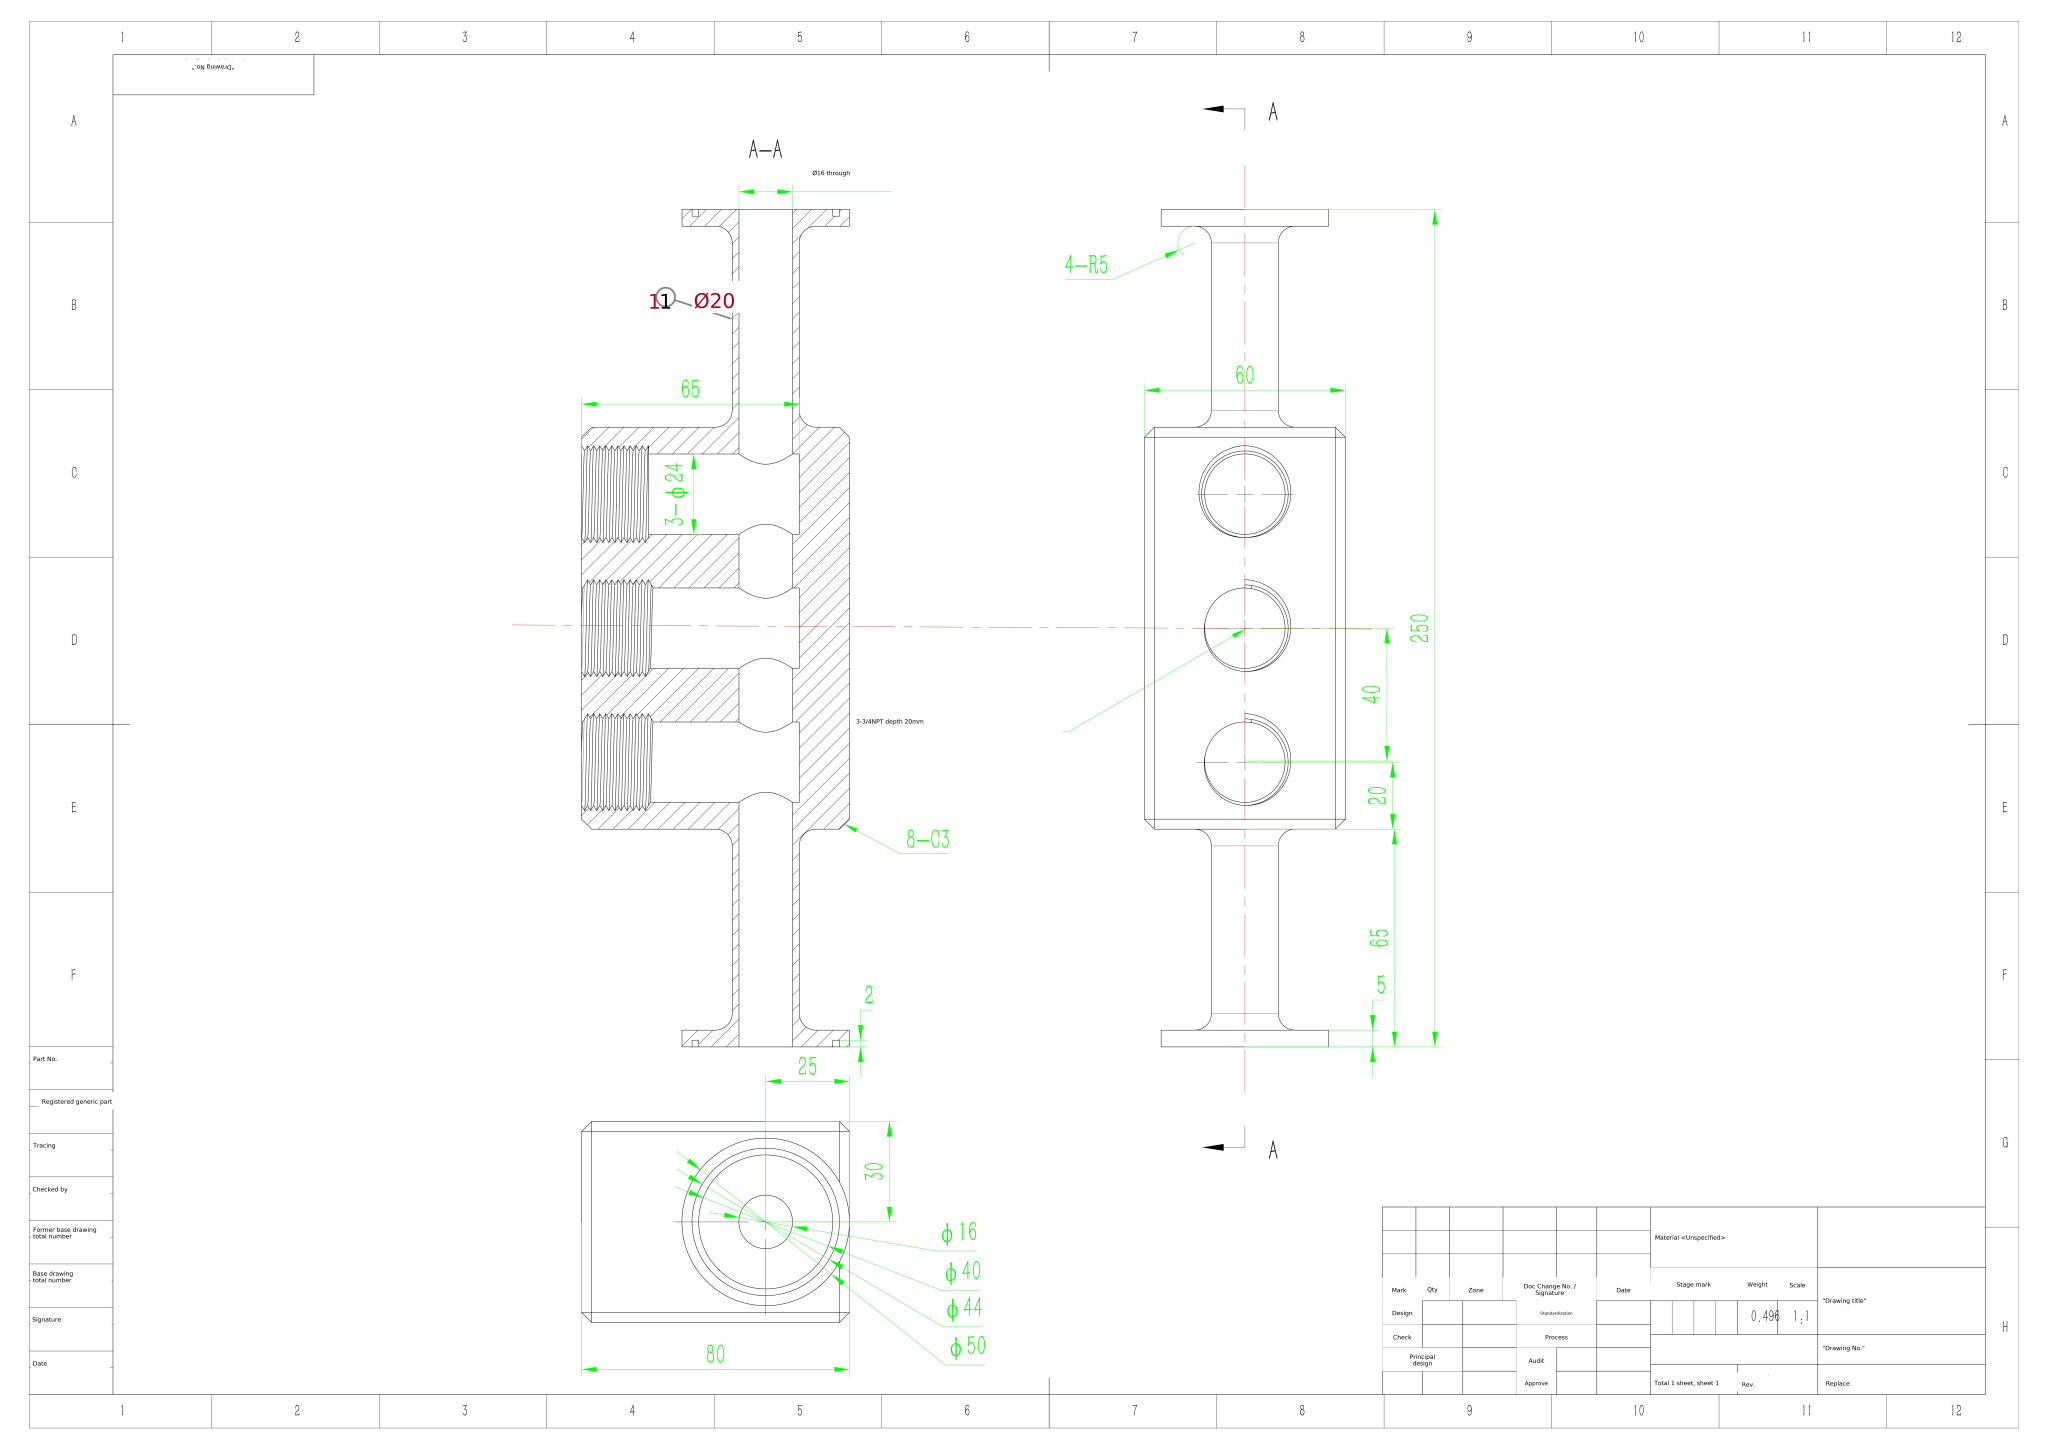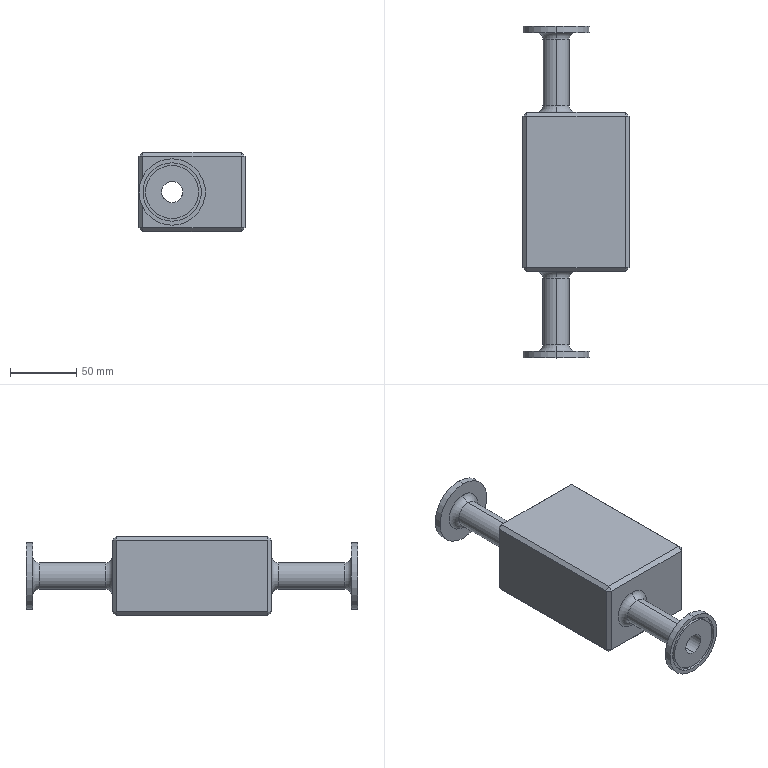Part | SolidWorks | mm | material <Unspecified> | 1 solid | 92 faces | box 80 x 250 x 60 mm | volume 496094 mm3 | plane 42 | cylinder 32 | spline 10 | torus 8 | commonest cylinder face diameters 16 x8 24 x8 40 x4 44 x4 50 x4 20 x4